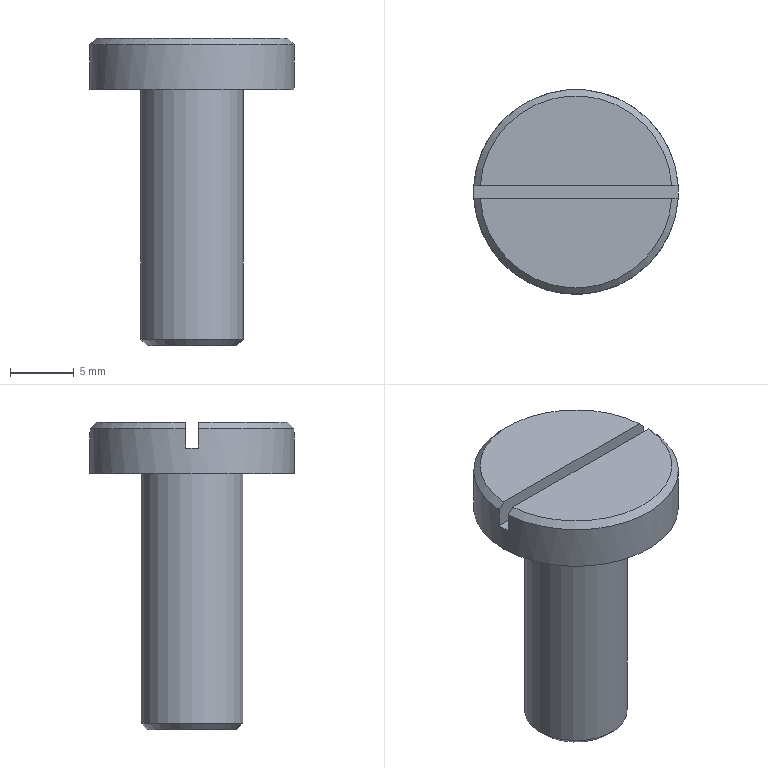Component | NX | DRILL_JIG_SCREW | 1 solid | 12 faces | box 16 x 16 x 24 mm | volume 1769 mm3 | plane 7 | cone 3 | cylinder 2 | commonest cylinder face diameters 16 x1 8 x1
STEP:
#1=CARTESIAN_POINT('',(0.,0.,0.));
#2=DIRECTION('',(0.,0.,1.));
#3=DIRECTION('',(1.,0.,0.));
#4=AXIS2_PLACEMENT_3D('',#1,#2,#3);
#5=CARTESIAN_POINT('',(-25.391,216.621,282.845));
#6=VERTEX_POINT('',#5);
#7=CARTESIAN_POINT('',(-10.425,216.621,282.845));
#8=VERTEX_POINT('',#7);
#9=CARTESIAN_POINT('',(-25.908,216.621,282.845));
#10=DIRECTION('',(1.,0.,0.));
#11=VECTOR('',#10,1.);
#12=LINE('',#9,#11);
#13=CARTESIAN_POINT('',(-17.908,216.121,282.845));
#14=DIRECTION('',(0.,0.,1.));
#15=DIRECTION('',(1.,0.,0.));
#16=AXIS2_PLACEMENT_3D('',#13,#14,#15);
#17=PLANE('',#16);
#18=CARTESIAN_POINT('',(-8.,0.5));
#19=DIRECTION('',(1.,0.));
#20=VECTOR('',#19,1.);
#21=LINE('',#18,#20);
#22=(GEOMETRIC_REPRESENTATION_CONTEXT(2)PARAMETRIC_REPRESENTATION_CONTEXT()REPRESENTATION_CONTEXT('',''));
#23=DEFINITIONAL_REPRESENTATION('',(#21),#22);
#24=PCURVE('',#17,#23);
#25=CARTESIAN_POINT('',(-25.908,216.621,282.845));
#26=DIRECTION('',(-0.,1.,0.));
#27=DIRECTION('',(1.,0.,0.));
#28=AXIS2_PLACEMENT_3D('',#25,#26,#27);
#29=PLANE('',#28);
#30=CARTESIAN_POINT('',(0.,0.));
#31=DIRECTION('',(1.,0.));
#32=VECTOR('',#31,1.);
#33=LINE('',#30,#32);
#34=(GEOMETRIC_REPRESENTATION_CONTEXT(2)PARAMETRIC_REPRESENTATION_CONTEXT()REPRESENTATION_CONTEXT('',''));
#35=DEFINITIONAL_REPRESENTATION('',(#33),#34);
#36=PCURVE('',#29,#35);
#37=SURFACE_CURVE('',#12,(#24,#36),.PCURVE_S1.);
#38=EDGE_CURVE('',#6,#8,#37,.T.);
#39=ORIENTED_EDGE('',*,*,#38,.T.);
#40=CARTESIAN_POINT('',(-17.908,216.121,282.845));
#41=DIRECTION('',(0.,0.,1.));
#42=DIRECTION('',(1.,0.,0.));
#43=AXIS2_PLACEMENT_3D('',#40,#41,#42);
#44=CIRCLE('',#43,7.5);
#45=CARTESIAN_POINT('',(0.,0.));
#46=DIRECTION('',(1.,0.));
#47=AXIS2_PLACEMENT_2D('',#45,#46);
#48=CIRCLE('',#47,7.5);
#49=(GEOMETRIC_REPRESENTATION_CONTEXT(2)PARAMETRIC_REPRESENTATION_CONTEXT()REPRESENTATION_CONTEXT('',''));
#50=DEFINITIONAL_REPRESENTATION('',(#48),#49);
#51=PCURVE('',#17,#50);
#52=CARTESIAN_POINT('',(-17.908,216.121,282.345));
#53=DIRECTION('',(0.,0.,-1.));
#54=DIRECTION('',(-1.,0.,0.));
#55=AXIS2_PLACEMENT_3D('',#52,#53,#54);
#56=CONICAL_SURFACE('',#55,8.,0.7854);
#57=CARTESIAN_POINT('',(3.142,-0.5));
#58=DIRECTION('',(-1.,0.));
#59=VECTOR('',#58,1.);
#60=LINE('',#57,#59);
#61=(GEOMETRIC_REPRESENTATION_CONTEXT(2)PARAMETRIC_REPRESENTATION_CONTEXT()REPRESENTATION_CONTEXT('',''));
#62=DEFINITIONAL_REPRESENTATION('',(#60),#61);
#63=PCURVE('',#56,#62);
#64=SURFACE_CURVE('',#44,(#51,#63),.PCURVE_S1.);
#65=EDGE_CURVE('',#8,#6,#64,.T.);
#66=ORIENTED_EDGE('',*,*,#65,.T.);
#67=EDGE_LOOP('',(#39,#66));
#68=FACE_BOUND('',#67,.T.);
#69=ADVANCED_FACE('',(#68),#17,.T.);
#70=CARTESIAN_POINT('',(-21.908,216.121,278.845));
#71=VERTEX_POINT('',#70);
#72=CARTESIAN_POINT('',(-17.908,216.121,278.845));
#73=DIRECTION('',(0.,0.,-1.));
#74=DIRECTION('',(-1.,0.,0.));
#75=AXIS2_PLACEMENT_3D('',#72,#73,#74);
#76=CIRCLE('',#75,4.);
#77=CARTESIAN_POINT('',(-17.908,216.121,278.845));
#78=DIRECTION('',(0.,0.,-1.));
#79=DIRECTION('',(-1.,0.,0.));
#80=AXIS2_PLACEMENT_3D('',#77,#78,#79);
#81=PLANE('',#80);
#82=CARTESIAN_POINT('',(0.,0.));
#83=DIRECTION('',(1.,0.));
#84=AXIS2_PLACEMENT_2D('',#82,#83);
#85=CIRCLE('',#84,4.);
#86=(GEOMETRIC_REPRESENTATION_CONTEXT(2)PARAMETRIC_REPRESENTATION_CONTEXT()REPRESENTATION_CONTEXT('',''));
#87=DEFINITIONAL_REPRESENTATION('',(#85),#86);
#88=PCURVE('',#81,#87);
#89=CARTESIAN_POINT('',(-17.908,216.121,278.845));
#90=DIRECTION('',(0.,0.,-1.));
#91=DIRECTION('',(-1.,0.,0.));
#92=AXIS2_PLACEMENT_3D('',#89,#90,#91);
#93=CYLINDRICAL_SURFACE('',#92,4.);
#94=CARTESIAN_POINT('',(0.,0.));
#95=DIRECTION('',(1.,0.));
#96=VECTOR('',#95,1.);
#97=LINE('',#94,#96);
#98=(GEOMETRIC_REPRESENTATION_CONTEXT(2)PARAMETRIC_REPRESENTATION_CONTEXT()REPRESENTATION_CONTEXT('',''));
#99=DEFINITIONAL_REPRESENTATION('',(#97),#98);
#100=PCURVE('',#93,#99);
#101=SURFACE_CURVE('',#76,(#88,#100),.PCURVE_S1.);
#102=EDGE_CURVE('',#71,#71,#101,.T.);
#103=ORIENTED_EDGE('',*,*,#102,.F.);
#104=EDGE_LOOP('',(#103));
#105=FACE_BOUND('',#104,.T.);
#106=CARTESIAN_POINT('',(-25.908,216.121,278.845));
#107=VERTEX_POINT('',#106);
#108=CARTESIAN_POINT('',(-17.908,216.121,278.845));
#109=DIRECTION('',(0.,0.,1.));
#110=DIRECTION('',(-1.,0.,0.));
#111=AXIS2_PLACEMENT_3D('',#108,#109,#110);
#112=CIRCLE('',#111,8.);
#113=CARTESIAN_POINT('',(8.,0.));
#114=CARTESIAN_POINT('',(8.,-13.856));
#115=CARTESIAN_POINT('',(-4.,-6.928));
#116=CARTESIAN_POINT('',(-16.,-0.));
#117=CARTESIAN_POINT('',(-4.,6.928));
#118=CARTESIAN_POINT('',(8.,13.856));
#119=CARTESIAN_POINT('',(8.,0.));
#120=(BOUNDED_CURVE()B_SPLINE_CURVE(2,(#113,#114,#115,#116,#117,#118,#119),.UNSPECIFIED.,.T.,.F.)B_SPLINE_CURVE_WITH_KNOTS((1,2,2,2,2,1),(-2.094,0.,2.094,4.189,6.283,8.378),.UNSPECIFIED.)CURVE()GEOMETRIC_REPRESENTATION_ITEM()RATIONAL_B_SPLINE_CURVE((1.,0.5,1.,0.5,1.,0.5,1.))REPRESENTATION_ITEM(''));
#121=(GEOMETRIC_REPRESENTATION_CONTEXT(2)PARAMETRIC_REPRESENTATION_CONTEXT()REPRESENTATION_CONTEXT('',''));
#122=DEFINITIONAL_REPRESENTATION('',(#120),#121);
#123=PCURVE('',#81,#122);
#124=CARTESIAN_POINT('',(-17.908,216.121,282.845));
#125=DIRECTION('',(0.,0.,-1.));
#126=DIRECTION('',(-1.,0.,0.));
#127=AXIS2_PLACEMENT_3D('',#124,#125,#126);
#128=CYLINDRICAL_SURFACE('',#127,8.);
#129=CARTESIAN_POINT('',(6.283,4.));
#130=DIRECTION('',(-1.,0.));
#131=VECTOR('',#130,1.);
#132=LINE('',#129,#131);
#133=(GEOMETRIC_REPRESENTATION_CONTEXT(2)PARAMETRIC_REPRESENTATION_CONTEXT()REPRESENTATION_CONTEXT('',''));
#134=DEFINITIONAL_REPRESENTATION('',(#132),#133);
#135=PCURVE('',#128,#134);
#136=SURFACE_CURVE('',#112,(#123,#135),.PCURVE_S1.);
#137=EDGE_CURVE('',#107,#107,#136,.T.);
#138=ORIENTED_EDGE('',*,*,#137,.F.);
#139=EDGE_LOOP('',(#138));
#140=FACE_BOUND('',#139,.T.);
#141=ADVANCED_FACE('',(#105,#140),#81,.T.);
#142=CARTESIAN_POINT('',(-25.391,215.621,282.845));
#143=VERTEX_POINT('',#142);
#144=CARTESIAN_POINT('',(-10.425,215.621,282.845));
#145=VERTEX_POINT('',#144);
#146=CARTESIAN_POINT('',(-25.908,215.621,282.845));
#147=DIRECTION('',(1.,0.,0.));
#148=VECTOR('',#147,1.);
#149=LINE('',#146,#148);
#150=CARTESIAN_POINT('',(-17.908,216.121,282.845));
#151=DIRECTION('',(0.,0.,1.));
#152=DIRECTION('',(1.,0.,0.));
#153=AXIS2_PLACEMENT_3D('',#150,#151,#152);
#154=PLANE('',#153);
#155=CARTESIAN_POINT('',(-8.,-0.5));
#156=DIRECTION('',(1.,0.));
#157=VECTOR('',#156,1.);
#158=LINE('',#155,#157);
#159=(GEOMETRIC_REPRESENTATION_CONTEXT(2)PARAMETRIC_REPRESENTATION_CONTEXT()REPRESENTATION_CONTEXT('',''));
#160=DEFINITIONAL_REPRESENTATION('',(#158),#159);
#161=PCURVE('',#154,#160);
#162=CARTESIAN_POINT('',(-25.908,215.621,282.845));
#163=DIRECTION('',(-0.,1.,0.));
#164=DIRECTION('',(1.,0.,0.));
#165=AXIS2_PLACEMENT_3D('',#162,#163,#164);
#166=PLANE('',#165);
#167=CARTESIAN_POINT('',(0.,0.));
#168=DIRECTION('',(1.,0.));
#169=VECTOR('',#168,1.);
#170=LINE('',#167,#169);
#171=(GEOMETRIC_REPRESENTATION_CONTEXT(2)PARAMETRIC_REPRESENTATION_CONTEXT()REPRESENTATION_CONTEXT('',''));
#172=DEFINITIONAL_REPRESENTATION('',(#170),#171);
#173=PCURVE('',#166,#172);
#174=SURFACE_CURVE('',#149,(#161,#173),.PCURVE_S1.);
#175=EDGE_CURVE('',#143,#145,#174,.T.);
#176=ORIENTED_EDGE('',*,*,#175,.F.);
#177=CARTESIAN_POINT('',(-17.908,216.121,282.845));
#178=DIRECTION('',(0.,0.,1.));
#179=DIRECTION('',(1.,0.,0.));
#180=AXIS2_PLACEMENT_3D('',#177,#178,#179);
#181=CIRCLE('',#180,7.5);
#182=CARTESIAN_POINT('',(0.,0.));
#183=DIRECTION('',(1.,0.));
#184=AXIS2_PLACEMENT_2D('',#182,#183);
#185=CIRCLE('',#184,7.5);
#186=(GEOMETRIC_REPRESENTATION_CONTEXT(2)PARAMETRIC_REPRESENTATION_CONTEXT()REPRESENTATION_CONTEXT('',''));
#187=DEFINITIONAL_REPRESENTATION('',(#185),#186);
#188=PCURVE('',#154,#187);
#189=CARTESIAN_POINT('',(-17.908,216.121,282.345));
#190=DIRECTION('',(0.,0.,-1.));
#191=DIRECTION('',(-1.,0.,0.));
#192=AXIS2_PLACEMENT_3D('',#189,#190,#191);
#193=CONICAL_SURFACE('',#192,8.,0.7854);
#194=CARTESIAN_POINT('',(9.425,-0.5));
#195=DIRECTION('',(-1.,0.));
#196=VECTOR('',#195,1.);
#197=LINE('',#194,#196);
#198=(GEOMETRIC_REPRESENTATION_CONTEXT(2)PARAMETRIC_REPRESENTATION_CONTEXT()REPRESENTATION_CONTEXT('',''));
#199=DEFINITIONAL_REPRESENTATION('',(#197),#198);
#200=PCURVE('',#193,#199);
#201=SURFACE_CURVE('',#181,(#188,#200),.PCURVE_S1.);
#202=EDGE_CURVE('',#143,#145,#201,.T.);
#203=ORIENTED_EDGE('',*,*,#202,.T.);
#204=EDGE_LOOP('',(#176,#203));
#205=FACE_BOUND('',#204,.T.);
#206=ADVANCED_FACE('',(#205),#154,.T.);
#207=CARTESIAN_POINT('',(-25.892,216.621,282.345));
#208=VERTEX_POINT('',#207);
#209=CARTESIAN_POINT('',(-25.892,216.621,280.845));
#210=VERTEX_POINT('',#209);
#211=CARTESIAN_POINT('',(-25.892,216.621,282.845));
#212=DIRECTION('',(0.,0.,-1.));
#213=VECTOR('',#212,1.);
#214=LINE('',#211,#213);
#215=CARTESIAN_POINT('',(0.06254,0.));
#216=DIRECTION('',(0.,1.));
#217=VECTOR('',#216,1.);
#218=LINE('',#215,#217);
#219=(GEOMETRIC_REPRESENTATION_CONTEXT(2)PARAMETRIC_REPRESENTATION_CONTEXT()REPRESENTATION_CONTEXT('',''));
#220=DEFINITIONAL_REPRESENTATION('',(#218),#219);
#221=PCURVE('',#128,#220);
#222=CARTESIAN_POINT('',(0.01564,0.));
#223=DIRECTION('',(0.,1.));
#224=VECTOR('',#223,1.);
#225=LINE('',#222,#224);
#226=(GEOMETRIC_REPRESENTATION_CONTEXT(2)PARAMETRIC_REPRESENTATION_CONTEXT()REPRESENTATION_CONTEXT('',''));
#227=DEFINITIONAL_REPRESENTATION('',(#225),#226);
#228=PCURVE('',#29,#227);
#229=SURFACE_CURVE('',#214,(#221,#228),.PCURVE_S1.);
#230=EDGE_CURVE('',#208,#210,#229,.T.);
#231=ORIENTED_EDGE('',*,*,#230,.F.);
#232=CARTESIAN_POINT('',(-9.924,216.621,282.345));
#233=VERTEX_POINT('',#232);
#234=CARTESIAN_POINT('',(-17.908,216.121,282.345));
#235=DIRECTION('',(0.,0.,-1.));
#236=DIRECTION('',(1.,0.,0.));
#237=AXIS2_PLACEMENT_3D('',#234,#235,#236);
#238=CIRCLE('',#237,8.);
#239=CARTESIAN_POINT('',(-3.142,0.5));
#240=DIRECTION('',(1.,0.));
#241=VECTOR('',#240,1.);
#242=LINE('',#239,#241);
#243=(GEOMETRIC_REPRESENTATION_CONTEXT(2)PARAMETRIC_REPRESENTATION_CONTEXT()REPRESENTATION_CONTEXT('',''));
#244=DEFINITIONAL_REPRESENTATION('',(#242),#243);
#245=PCURVE('',#128,#244);
#246=CARTESIAN_POINT('',(-3.142,0.));
#247=DIRECTION('',(1.,0.));
#248=VECTOR('',#247,1.);
#249=LINE('',#246,#248);
#250=(GEOMETRIC_REPRESENTATION_CONTEXT(2)PARAMETRIC_REPRESENTATION_CONTEXT()REPRESENTATION_CONTEXT('',''));
#251=DEFINITIONAL_REPRESENTATION('',(#249),#250);
#252=PCURVE('',#56,#251);
#253=SURFACE_CURVE('',#238,(#245,#252),.PCURVE_S1.);
#254=EDGE_CURVE('',#208,#233,#253,.T.);
#255=ORIENTED_EDGE('',*,*,#254,.T.);
#256=CARTESIAN_POINT('',(-9.924,216.621,280.845));
#257=VERTEX_POINT('',#256);
#258=CARTESIAN_POINT('',(-9.924,216.621,282.845));
#259=DIRECTION('',(0.,0.,1.));
#260=VECTOR('',#259,1.);
#261=LINE('',#258,#260);
#262=CARTESIAN_POINT('',(3.079,0.));
#263=DIRECTION('',(0.,-1.));
#264=VECTOR('',#263,1.);
#265=LINE('',#262,#264);
#266=(GEOMETRIC_REPRESENTATION_CONTEXT(2)PARAMETRIC_REPRESENTATION_CONTEXT()REPRESENTATION_CONTEXT('',''));
#267=DEFINITIONAL_REPRESENTATION('',(#265),#266);
#268=PCURVE('',#128,#267);
#269=CARTESIAN_POINT('',(15.984,0.));
#270=DIRECTION('',(0.,-1.));
#271=VECTOR('',#270,1.);
#272=LINE('',#269,#271);
#273=(GEOMETRIC_REPRESENTATION_CONTEXT(2)PARAMETRIC_REPRESENTATION_CONTEXT()REPRESENTATION_CONTEXT('',''));
#274=DEFINITIONAL_REPRESENTATION('',(#272),#273);
#275=PCURVE('',#29,#274);
#276=SURFACE_CURVE('',#261,(#268,#275),.PCURVE_S1.);
#277=EDGE_CURVE('',#257,#233,#276,.T.);
#278=ORIENTED_EDGE('',*,*,#277,.F.);
#279=CARTESIAN_POINT('',(-9.924,215.621,280.845));
#280=VERTEX_POINT('',#279);
#281=CARTESIAN_POINT('',(-17.908,216.121,280.845));
#282=DIRECTION('',(0.,0.,1.));
#283=DIRECTION('',(1.,0.,0.));
#284=AXIS2_PLACEMENT_3D('',#281,#282,#283);
#285=CIRCLE('',#284,8.);
#286=CARTESIAN_POINT('',(9.425,2.));
#287=DIRECTION('',(-1.,0.));
#288=VECTOR('',#287,1.);
#289=LINE('',#286,#288);
#290=(GEOMETRIC_REPRESENTATION_CONTEXT(2)PARAMETRIC_REPRESENTATION_CONTEXT()REPRESENTATION_CONTEXT('',''));
#291=DEFINITIONAL_REPRESENTATION('',(#289),#290);
#292=PCURVE('',#128,#291);
#293=CARTESIAN_POINT('',(-25.908,216.121,280.845));
#294=DIRECTION('',(0.,0.,1.));
#295=DIRECTION('',(1.,0.,0.));
#296=AXIS2_PLACEMENT_3D('',#293,#294,#295);
#297=PLANE('',#296);
#298=CARTESIAN_POINT('',(8.,-0.));
#299=DIRECTION('',(1.,-0.));
#300=AXIS2_PLACEMENT_2D('',#298,#299);
#301=CIRCLE('',#300,8.);
#302=(GEOMETRIC_REPRESENTATION_CONTEXT(2)PARAMETRIC_REPRESENTATION_CONTEXT()REPRESENTATION_CONTEXT('',''));
#303=DEFINITIONAL_REPRESENTATION('',(#301),#302);
#304=PCURVE('',#297,#303);
#305=SURFACE_CURVE('',#285,(#292,#304),.PCURVE_S1.);
#306=EDGE_CURVE('',#280,#257,#305,.T.);
#307=ORIENTED_EDGE('',*,*,#306,.F.);
#308=CARTESIAN_POINT('',(-9.924,215.621,282.345));
#309=VERTEX_POINT('',#308);
#310=CARTESIAN_POINT('',(-9.924,215.621,282.845));
#311=DIRECTION('',(0.,0.,1.));
#312=VECTOR('',#311,1.);
#313=LINE('',#310,#312);
#314=CARTESIAN_POINT('',(3.204,0.));
#315=DIRECTION('',(0.,-1.));
#316=VECTOR('',#315,1.);
#317=LINE('',#314,#316);
#318=(GEOMETRIC_REPRESENTATION_CONTEXT(2)PARAMETRIC_REPRESENTATION_CONTEXT()REPRESENTATION_CONTEXT('',''));
#319=DEFINITIONAL_REPRESENTATION('',(#317),#318);
#320=PCURVE('',#128,#319);
#321=CARTESIAN_POINT('',(15.984,0.));
#322=DIRECTION('',(0.,-1.));
#323=VECTOR('',#322,1.);
#324=LINE('',#321,#323);
#325=(GEOMETRIC_REPRESENTATION_CONTEXT(2)PARAMETRIC_REPRESENTATION_CONTEXT()REPRESENTATION_CONTEXT('',''));
#326=DEFINITIONAL_REPRESENTATION('',(#324),#325);
#327=PCURVE('',#166,#326);
#328=SURFACE_CURVE('',#313,(#320,#327),.PCURVE_S1.);
#329=EDGE_CURVE('',#280,#309,#328,.T.);
#330=ORIENTED_EDGE('',*,*,#329,.T.);
#331=CARTESIAN_POINT('',(-25.892,215.621,282.345));
#332=VERTEX_POINT('',#331);
#333=CARTESIAN_POINT('',(-17.908,216.121,282.345));
#334=DIRECTION('',(0.,0.,-1.));
#335=DIRECTION('',(1.,0.,0.));
#336=AXIS2_PLACEMENT_3D('',#333,#334,#335);
#337=CIRCLE('',#336,8.);
#338=CARTESIAN_POINT('',(3.142,0.5));
#339=DIRECTION('',(1.,0.));
#340=VECTOR('',#339,1.);
#341=LINE('',#338,#340);
#342=(GEOMETRIC_REPRESENTATION_CONTEXT(2)PARAMETRIC_REPRESENTATION_CONTEXT()REPRESENTATION_CONTEXT('',''));
#343=DEFINITIONAL_REPRESENTATION('',(#341),#342);
#344=PCURVE('',#128,#343);
#345=CARTESIAN_POINT('',(3.142,0.));
#346=DIRECTION('',(1.,0.));
#347=VECTOR('',#346,1.);
#348=LINE('',#345,#347);
#349=(GEOMETRIC_REPRESENTATION_CONTEXT(2)PARAMETRIC_REPRESENTATION_CONTEXT()REPRESENTATION_CONTEXT('',''));
#350=DEFINITIONAL_REPRESENTATION('',(#348),#349);
#351=PCURVE('',#193,#350);
#352=SURFACE_CURVE('',#337,(#344,#351),.PCURVE_S1.);
#353=EDGE_CURVE('',#309,#332,#352,.T.);
#354=ORIENTED_EDGE('',*,*,#353,.T.);
#355=CARTESIAN_POINT('',(-25.892,215.621,280.845));
#356=VERTEX_POINT('',#355);
#357=CARTESIAN_POINT('',(-25.892,215.621,282.845));
#358=DIRECTION('',(0.,0.,-1.));
#359=VECTOR('',#358,1.);
#360=LINE('',#357,#359);
#361=CARTESIAN_POINT('',(6.221,0.));
#362=DIRECTION('',(0.,1.));
#363=VECTOR('',#362,1.);
#364=LINE('',#361,#363);
#365=(GEOMETRIC_REPRESENTATION_CONTEXT(2)PARAMETRIC_REPRESENTATION_CONTEXT()REPRESENTATION_CONTEXT('',''));
#366=DEFINITIONAL_REPRESENTATION('',(#364),#365);
#367=PCURVE('',#128,#366);
#368=CARTESIAN_POINT('',(0.01564,0.));
#369=DIRECTION('',(0.,1.));
#370=VECTOR('',#369,1.);
#371=LINE('',#368,#370);
#372=(GEOMETRIC_REPRESENTATION_CONTEXT(2)PARAMETRIC_REPRESENTATION_CONTEXT()REPRESENTATION_CONTEXT('',''));
#373=DEFINITIONAL_REPRESENTATION('',(#371),#372);
#374=PCURVE('',#166,#373);
#375=SURFACE_CURVE('',#360,(#367,#374),.PCURVE_S1.);
#376=EDGE_CURVE('',#332,#356,#375,.T.);
#377=ORIENTED_EDGE('',*,*,#376,.T.);
#378=CARTESIAN_POINT('',(-25.908,216.121,280.845));
#379=VERTEX_POINT('',#378);
#380=CARTESIAN_POINT('',(-17.908,216.121,280.845));
#381=DIRECTION('',(0.,0.,1.));
#382=DIRECTION('',(1.,0.,0.));
#383=AXIS2_PLACEMENT_3D('',#380,#381,#382);
#384=CIRCLE('',#383,8.);
#385=CARTESIAN_POINT('',(9.425,2.));
#386=DIRECTION('',(-1.,0.));
#387=VECTOR('',#386,1.);
#388=LINE('',#385,#387);
#389=(GEOMETRIC_REPRESENTATION_CONTEXT(2)PARAMETRIC_REPRESENTATION_CONTEXT()REPRESENTATION_CONTEXT('',''));
#390=DEFINITIONAL_REPRESENTATION('',(#388),#389);
#391=PCURVE('',#128,#390);
#392=CARTESIAN_POINT('',(8.,-0.));
#393=DIRECTION('',(1.,-0.));
#394=AXIS2_PLACEMENT_2D('',#392,#393);
#395=CIRCLE('',#394,8.);
#396=(GEOMETRIC_REPRESENTATION_CONTEXT(2)PARAMETRIC_REPRESENTATION_CONTEXT()REPRESENTATION_CONTEXT('',''));
#397=DEFINITIONAL_REPRESENTATION('',(#395),#396);
#398=PCURVE('',#297,#397);
#399=SURFACE_CURVE('',#384,(#391,#398),.PCURVE_S1.);
#400=EDGE_CURVE('',#379,#356,#399,.T.);
#401=ORIENTED_EDGE('',*,*,#400,.F.);
#402=CARTESIAN_POINT('',(-25.908,216.121,280.845));
#403=CARTESIAN_POINT('',(-25.908,216.121,278.845));
#404=B_SPLINE_CURVE_WITH_KNOTS('',1,(#402,#403),.UNSPECIFIED.,.F.,.F.,(2,2),(2.,4.),.PIECEWISE_BEZIER_KNOTS.);
#405=CARTESIAN_POINT('',(6.283,0.));
#406=DIRECTION('',(0.,1.));
#407=VECTOR('',#406,1.);
#408=LINE('',#405,#407);
#409=(GEOMETRIC_REPRESENTATION_CONTEXT(2)PARAMETRIC_REPRESENTATION_CONTEXT()REPRESENTATION_CONTEXT('',''));
#410=DEFINITIONAL_REPRESENTATION('',(#408),#409);
#411=PCURVE('',#128,#410);
#412=CARTESIAN_POINT('',(0.,0.));
#413=DIRECTION('',(0.,1.));
#414=VECTOR('',#413,1.);
#415=LINE('',#412,#414);
#416=(GEOMETRIC_REPRESENTATION_CONTEXT(2)PARAMETRIC_REPRESENTATION_CONTEXT()REPRESENTATION_CONTEXT('',''));
#417=DEFINITIONAL_REPRESENTATION('',(#415),#416);
#418=PCURVE('',#128,#417);
#419=SEAM_CURVE('',#404,(#411,#418),.PCURVE_S1.);
#420=EDGE_CURVE('',#379,#107,#419,.T.);
#421=ORIENTED_EDGE('',*,*,#420,.T.);
#422=ORIENTED_EDGE('',*,*,#137,.T.);
#423=ORIENTED_EDGE('',*,*,#420,.F.);
#424=CARTESIAN_POINT('',(-17.908,216.121,280.845));
#425=DIRECTION('',(0.,0.,1.));
#426=DIRECTION('',(1.,0.,0.));
#427=AXIS2_PLACEMENT_3D('',#424,#425,#426);
#428=CIRCLE('',#427,8.);
#429=CARTESIAN_POINT('',(3.142,2.));
#430=DIRECTION('',(-1.,0.));
#431=VECTOR('',#430,1.);
#432=LINE('',#429,#431);
#433=(GEOMETRIC_REPRESENTATION_CONTEXT(2)PARAMETRIC_REPRESENTATION_CONTEXT()REPRESENTATION_CONTEXT('',''));
#434=DEFINITIONAL_REPRESENTATION('',(#432),#433);
#435=PCURVE('',#128,#434);
#436=CARTESIAN_POINT('',(8.,-0.));
#437=DIRECTION('',(1.,-0.));
#438=AXIS2_PLACEMENT_2D('',#436,#437);
#439=CIRCLE('',#438,8.);
#440=(GEOMETRIC_REPRESENTATION_CONTEXT(2)PARAMETRIC_REPRESENTATION_CONTEXT()REPRESENTATION_CONTEXT('',''));
#441=DEFINITIONAL_REPRESENTATION('',(#439),#440);
#442=PCURVE('',#297,#441);
#443=SURFACE_CURVE('',#428,(#435,#442),.PCURVE_S1.);
#444=EDGE_CURVE('',#210,#379,#443,.T.);
#445=ORIENTED_EDGE('',*,*,#444,.F.);
#446=EDGE_LOOP('',(#231,#255,#278,#307,#330,#354,#377,#401,#421,#422,#423,#445));
#447=FACE_BOUND('',#446,.T.);
#448=ADVANCED_FACE('',(#447),#128,.T.);
#449=CARTESIAN_POINT('',(-21.408,216.121,258.845));
#450=VERTEX_POINT('',#449);
#451=CARTESIAN_POINT('',(-17.908,216.121,258.845));
#452=DIRECTION('',(0.,0.,-1.));
#453=DIRECTION('',(-1.,0.,0.));
#454=AXIS2_PLACEMENT_3D('',#451,#452,#453);
#455=CIRCLE('',#454,3.5);
#456=CARTESIAN_POINT('',(-17.908,216.121,258.845));
#457=DIRECTION('',(0.,0.,-1.));
#458=DIRECTION('',(-1.,0.,0.));
#459=AXIS2_PLACEMENT_3D('',#456,#457,#458);
#460=PLANE('',#459);
#461=CARTESIAN_POINT('',(0.,0.));
#462=DIRECTION('',(1.,0.));
#463=AXIS2_PLACEMENT_2D('',#461,#462);
#464=CIRCLE('',#463,3.5);
#465=(GEOMETRIC_REPRESENTATION_CONTEXT(2)PARAMETRIC_REPRESENTATION_CONTEXT()REPRESENTATION_CONTEXT('',''));
#466=DEFINITIONAL_REPRESENTATION('',(#464),#465);
#467=PCURVE('',#460,#466);
#468=CARTESIAN_POINT('',(-17.908,216.121,259.345));
#469=DIRECTION('',(0.,0.,1.));
#470=DIRECTION('',(1.,0.,0.));
#471=AXIS2_PLACEMENT_3D('',#468,#469,#470);
#472=CONICAL_SURFACE('',#471,4.,0.7854);
#473=CARTESIAN_POINT('',(9.425,-0.5));
#474=DIRECTION('',(-1.,0.));
#475=VECTOR('',#474,1.);
#476=LINE('',#473,#475);
#477=(GEOMETRIC_REPRESENTATION_CONTEXT(2)PARAMETRIC_REPRESENTATION_CONTEXT()REPRESENTATION_CONTEXT('',''));
#478=DEFINITIONAL_REPRESENTATION('',(#476),#477);
#479=PCURVE('',#472,#478);
#480=SURFACE_CURVE('',#455,(#467,#479),.PCURVE_S1.);
#481=EDGE_CURVE('',#450,#450,#480,.T.);
#482=ORIENTED_EDGE('',*,*,#481,.T.);
#483=EDGE_LOOP('',(#482));
#484=FACE_BOUND('',#483,.T.);
#485=ADVANCED_FACE('',(#484),#460,.T.);
#486=CARTESIAN_POINT('',(-21.908,216.121,259.345));
#487=VERTEX_POINT('',#486);
#488=CARTESIAN_POINT('',(-17.908,216.121,259.345));
#489=DIRECTION('',(0.,0.,1.));
#490=DIRECTION('',(-1.,0.,0.));
#491=AXIS2_PLACEMENT_3D('',#488,#489,#490);
#492=CIRCLE('',#491,4.);
#493=CARTESIAN_POINT('',(6.283,19.5));
#494=DIRECTION('',(-1.,0.));
#495=VECTOR('',#494,1.);
#496=LINE('',#493,#495);
#497=(GEOMETRIC_REPRESENTATION_CONTEXT(2)PARAMETRIC_REPRESENTATION_CONTEXT()REPRESENTATION_CONTEXT('',''));
#498=DEFINITIONAL_REPRESENTATION('',(#496),#497);
#499=PCURVE('',#93,#498);
#500=CARTESIAN_POINT('',(3.142,0.));
#501=DIRECTION('',(1.,0.));
#502=VECTOR('',#501,1.);
#503=LINE('',#500,#502);
#504=(GEOMETRIC_REPRESENTATION_CONTEXT(2)PARAMETRIC_REPRESENTATION_CONTEXT()REPRESENTATION_CONTEXT('',''));
#505=DEFINITIONAL_REPRESENTATION('',(#503),#504);
#506=PCURVE('',#472,#505);
#507=SURFACE_CURVE('',#492,(#499,#506),.PCURVE_S1.);
#508=EDGE_CURVE('',#487,#487,#507,.T.);
#509=ORIENTED_EDGE('',*,*,#508,.T.);
#510=CARTESIAN_POINT('',(-21.908,216.121,278.845));
#511=CARTESIAN_POINT('',(-21.908,216.121,259.345));
#512=B_SPLINE_CURVE_WITH_KNOTS('',1,(#510,#511),.UNSPECIFIED.,.F.,.F.,(2,2),(0.,19.5),.PIECEWISE_BEZIER_KNOTS.);
#513=CARTESIAN_POINT('',(0.,0.));
#514=DIRECTION('',(0.,1.));
#515=VECTOR('',#514,1.);
#516=LINE('',#513,#515);
#517=(GEOMETRIC_REPRESENTATION_CONTEXT(2)PARAMETRIC_REPRESENTATION_CONTEXT()REPRESENTATION_CONTEXT('',''));
#518=DEFINITIONAL_REPRESENTATION('',(#516),#517);
#519=PCURVE('',#93,#518);
#520=CARTESIAN_POINT('',(6.283,0.));
#521=DIRECTION('',(0.,1.));
#522=VECTOR('',#521,1.);
#523=LINE('',#520,#522);
#524=(GEOMETRIC_REPRESENTATION_CONTEXT(2)PARAMETRIC_REPRESENTATION_CONTEXT()REPRESENTATION_CONTEXT('',''));
#525=DEFINITIONAL_REPRESENTATION('',(#523),#524);
#526=PCURVE('',#93,#525);
#527=SEAM_CURVE('',#512,(#519,#526),.PCURVE_S1.);
#528=EDGE_CURVE('',#71,#487,#527,.T.);
#529=ORIENTED_EDGE('',*,*,#528,.F.);
#530=ORIENTED_EDGE('',*,*,#102,.T.);
#531=ORIENTED_EDGE('',*,*,#528,.T.);
#532=EDGE_LOOP('',(#509,#529,#530,#531));
#533=FACE_BOUND('',#532,.T.);
#534=ADVANCED_FACE('',(#533),#93,.T.);
#535=CARTESIAN_POINT('',(-25.908,216.621,280.845));
#536=DIRECTION('',(-1.,-0.,0.));
#537=VECTOR('',#536,1.);
#538=LINE('',#535,#537);
#539=CARTESIAN_POINT('',(0.,0.5));
#540=DIRECTION('',(-1.,-0.));
#541=VECTOR('',#540,1.);
#542=LINE('',#539,#541);
#543=(GEOMETRIC_REPRESENTATION_CONTEXT(2)PARAMETRIC_REPRESENTATION_CONTEXT()REPRESENTATION_CONTEXT('',''));
#544=DEFINITIONAL_REPRESENTATION('',(#542),#543);
#545=PCURVE('',#297,#544);
#546=CARTESIAN_POINT('',(0.,2.));
#547=DIRECTION('',(-1.,0.));
#548=VECTOR('',#547,1.);
#549=LINE('',#546,#548);
#550=(GEOMETRIC_REPRESENTATION_CONTEXT(2)PARAMETRIC_REPRESENTATION_CONTEXT()REPRESENTATION_CONTEXT('',''));
#551=DEFINITIONAL_REPRESENTATION('',(#549),#550);
#552=PCURVE('',#29,#551);
#553=SURFACE_CURVE('',#538,(#545,#552),.PCURVE_S1.);
#554=EDGE_CURVE('',#257,#210,#553,.T.);
#555=ORIENTED_EDGE('',*,*,#554,.T.);
#556=ORIENTED_EDGE('',*,*,#444,.T.);
#557=ORIENTED_EDGE('',*,*,#400,.T.);
#558=CARTESIAN_POINT('',(-25.908,215.621,280.845));
#559=DIRECTION('',(-1.,-0.,0.));
#560=VECTOR('',#559,1.);
#561=LINE('',#558,#560);
#562=CARTESIAN_POINT('',(-0.,-0.5));
#563=DIRECTION('',(-1.,-0.));
#564=VECTOR('',#563,1.);
#565=LINE('',#562,#564);
#566=(GEOMETRIC_REPRESENTATION_CONTEXT(2)PARAMETRIC_REPRESENTATION_CONTEXT()REPRESENTATION_CONTEXT('',''));
#567=DEFINITIONAL_REPRESENTATION('',(#565),#566);
#568=PCURVE('',#297,#567);
#569=CARTESIAN_POINT('',(0.,2.));
#570=DIRECTION('',(-1.,0.));
#571=VECTOR('',#570,1.);
#572=LINE('',#569,#571);
#573=(GEOMETRIC_REPRESENTATION_CONTEXT(2)PARAMETRIC_REPRESENTATION_CONTEXT()REPRESENTATION_CONTEXT('',''));
#574=DEFINITIONAL_REPRESENTATION('',(#572),#573);
#575=PCURVE('',#166,#574);
#576=SURFACE_CURVE('',#561,(#568,#575),.PCURVE_S1.);
#577=EDGE_CURVE('',#280,#356,#576,.T.);
#578=ORIENTED_EDGE('',*,*,#577,.F.);
#579=ORIENTED_EDGE('',*,*,#306,.T.);
#580=EDGE_LOOP('',(#555,#556,#557,#578,#579));
#581=FACE_BOUND('',#580,.T.);
#582=ADVANCED_FACE('',(#581),#297,.T.);
#583=ORIENTED_EDGE('',*,*,#277,.T.);
#584=CARTESIAN_POINT('',(-9.924,216.621,282.345));
#585=CARTESIAN_POINT('',(-10.091,216.621,282.511));
#586=CARTESIAN_POINT('',(-10.258,216.621,282.678));
#587=CARTESIAN_POINT('',(-10.425,216.621,282.845));
#588=B_SPLINE_CURVE_WITH_KNOTS('',3,(#584,#585,#586,#587),.UNSPECIFIED.,.F.,.F.,(4,4),(0.,1.),.PIECEWISE_BEZIER_KNOTS.);
#589=CARTESIAN_POINT('',(15.984,0.5));
#590=CARTESIAN_POINT('',(15.817,0.3333));
#591=CARTESIAN_POINT('',(15.65,0.1667));
#592=CARTESIAN_POINT('',(15.483,0.));
#593=B_SPLINE_CURVE_WITH_KNOTS('',3,(#589,#590,#591,#592),.UNSPECIFIED.,.F.,.F.,(4,4),(0.,1.),.PIECEWISE_BEZIER_KNOTS.);
#594=(GEOMETRIC_REPRESENTATION_CONTEXT(2)PARAMETRIC_REPRESENTATION_CONTEXT()REPRESENTATION_CONTEXT('',''));
#595=DEFINITIONAL_REPRESENTATION('',(#593),#594);
#596=PCURVE('',#29,#595);
#597=CARTESIAN_POINT('',(3.079,-0.));
#598=CARTESIAN_POINT('',(3.075,-0.5));
#599=B_SPLINE_CURVE_WITH_KNOTS('',1,(#597,#598),.UNSPECIFIED.,.F.,.F.,(2,2),(0.,1.),.PIECEWISE_BEZIER_KNOTS.);
#600=(GEOMETRIC_REPRESENTATION_CONTEXT(2)PARAMETRIC_REPRESENTATION_CONTEXT()REPRESENTATION_CONTEXT('',''));
#601=DEFINITIONAL_REPRESENTATION('',(#599),#600);
#602=PCURVE('',#56,#601);
#603=SURFACE_CURVE('',#588,(#596,#602),.PCURVE_S1.);
#604=EDGE_CURVE('',#233,#8,#603,.T.);
#605=ORIENTED_EDGE('',*,*,#604,.T.);
#606=ORIENTED_EDGE('',*,*,#38,.F.);
#607=CARTESIAN_POINT('',(-25.391,216.621,282.845));
#608=CARTESIAN_POINT('',(-25.558,216.621,282.678));
#609=CARTESIAN_POINT('',(-25.725,216.621,282.511));
#610=CARTESIAN_POINT('',(-25.892,216.621,282.345));
#611=B_SPLINE_CURVE_WITH_KNOTS('',3,(#607,#608,#609,#610),.UNSPECIFIED.,.F.,.F.,(4,4),(0.,1.),.PIECEWISE_BEZIER_KNOTS.);
#612=CARTESIAN_POINT('',(0.5167,0.));
#613=CARTESIAN_POINT('',(0.3497,0.1667));
#614=CARTESIAN_POINT('',(0.1826,0.3333));
#615=CARTESIAN_POINT('',(0.01564,0.5));
#616=B_SPLINE_CURVE_WITH_KNOTS('',3,(#612,#613,#614,#615),.UNSPECIFIED.,.F.,.F.,(4,4),(0.,1.),.PIECEWISE_BEZIER_KNOTS.);
#617=(GEOMETRIC_REPRESENTATION_CONTEXT(2)PARAMETRIC_REPRESENTATION_CONTEXT()REPRESENTATION_CONTEXT('',''));
#618=DEFINITIONAL_REPRESENTATION('',(#616),#617);
#619=PCURVE('',#29,#618);
#620=CARTESIAN_POINT('',(0.06672,-0.5));
#621=CARTESIAN_POINT('',(0.06254,0.));
#622=B_SPLINE_CURVE_WITH_KNOTS('',1,(#620,#621),.UNSPECIFIED.,.F.,.F.,(2,2),(0.,1.),.PIECEWISE_BEZIER_KNOTS.);
#623=(GEOMETRIC_REPRESENTATION_CONTEXT(2)PARAMETRIC_REPRESENTATION_CONTEXT()REPRESENTATION_CONTEXT('',''));
#624=DEFINITIONAL_REPRESENTATION('',(#622),#623);
#625=PCURVE('',#56,#624);
#626=SURFACE_CURVE('',#611,(#619,#625),.PCURVE_S1.);
#627=EDGE_CURVE('',#6,#208,#626,.T.);
#628=ORIENTED_EDGE('',*,*,#627,.T.);
#629=ORIENTED_EDGE('',*,*,#230,.T.);
#630=ORIENTED_EDGE('',*,*,#554,.F.);
#631=EDGE_LOOP('',(#583,#605,#606,#628,#629,#630));
#632=FACE_BOUND('',#631,.T.);
#633=ADVANCED_FACE('',(#632),#29,.F.);
#634=ORIENTED_EDGE('',*,*,#376,.F.);
#635=CARTESIAN_POINT('',(-25.892,215.621,282.345));
#636=CARTESIAN_POINT('',(-25.725,215.621,282.511));
#637=CARTESIAN_POINT('',(-25.558,215.621,282.678));
#638=CARTESIAN_POINT('',(-25.391,215.621,282.845));
#639=B_SPLINE_CURVE_WITH_KNOTS('',3,(#635,#636,#637,#638),.UNSPECIFIED.,.F.,.F.,(4,4),(0.,1.),.PIECEWISE_BEZIER_KNOTS.);
#640=CARTESIAN_POINT('',(0.01564,0.5));
#641=CARTESIAN_POINT('',(0.1826,0.3333));
#642=CARTESIAN_POINT('',(0.3497,0.1667));
#643=CARTESIAN_POINT('',(0.5167,0.));
#644=B_SPLINE_CURVE_WITH_KNOTS('',3,(#640,#641,#642,#643),.UNSPECIFIED.,.F.,.F.,(4,4),(0.,1.),.PIECEWISE_BEZIER_KNOTS.);
#645=(GEOMETRIC_REPRESENTATION_CONTEXT(2)PARAMETRIC_REPRESENTATION_CONTEXT()REPRESENTATION_CONTEXT('',''));
#646=DEFINITIONAL_REPRESENTATION('',(#644),#645);
#647=PCURVE('',#166,#646);
#648=CARTESIAN_POINT('',(6.221,0.));
#649=CARTESIAN_POINT('',(6.216,-0.5));
#650=B_SPLINE_CURVE_WITH_KNOTS('',1,(#648,#649),.UNSPECIFIED.,.F.,.F.,(2,2),(0.,1.),.PIECEWISE_BEZIER_KNOTS.);
#651=(GEOMETRIC_REPRESENTATION_CONTEXT(2)PARAMETRIC_REPRESENTATION_CONTEXT()REPRESENTATION_CONTEXT('',''));
#652=DEFINITIONAL_REPRESENTATION('',(#650),#651);
#653=PCURVE('',#193,#652);
#654=SURFACE_CURVE('',#639,(#647,#653),.PCURVE_S1.);
#655=EDGE_CURVE('',#332,#143,#654,.T.);
#656=ORIENTED_EDGE('',*,*,#655,.T.);
#657=ORIENTED_EDGE('',*,*,#175,.T.);
#658=CARTESIAN_POINT('',(-10.425,215.621,282.845));
#659=CARTESIAN_POINT('',(-10.258,215.621,282.678));
#660=CARTESIAN_POINT('',(-10.091,215.621,282.511));
#661=CARTESIAN_POINT('',(-9.924,215.621,282.345));
#662=B_SPLINE_CURVE_WITH_KNOTS('',3,(#658,#659,#660,#661),.UNSPECIFIED.,.F.,.F.,(4,4),(0.,1.),.PIECEWISE_BEZIER_KNOTS.);
#663=CARTESIAN_POINT('',(15.483,0.));
#664=CARTESIAN_POINT('',(15.65,0.1667));
#665=CARTESIAN_POINT('',(15.817,0.3333));
#666=CARTESIAN_POINT('',(15.984,0.5));
#667=B_SPLINE_CURVE_WITH_KNOTS('',3,(#663,#664,#665,#666),.UNSPECIFIED.,.F.,.F.,(4,4),(0.,1.),.PIECEWISE_BEZIER_KNOTS.);
#668=(GEOMETRIC_REPRESENTATION_CONTEXT(2)PARAMETRIC_REPRESENTATION_CONTEXT()REPRESENTATION_CONTEXT('',''));
#669=DEFINITIONAL_REPRESENTATION('',(#667),#668);
#670=PCURVE('',#166,#669);
#671=CARTESIAN_POINT('',(3.208,-0.5));
#672=CARTESIAN_POINT('',(3.204,-0.));
#673=B_SPLINE_CURVE_WITH_KNOTS('',1,(#671,#672),.UNSPECIFIED.,.F.,.F.,(2,2),(0.,1.),.PIECEWISE_BEZIER_KNOTS.);
#674=(GEOMETRIC_REPRESENTATION_CONTEXT(2)PARAMETRIC_REPRESENTATION_CONTEXT()REPRESENTATION_CONTEXT('',''));
#675=DEFINITIONAL_REPRESENTATION('',(#673),#674);
#676=PCURVE('',#193,#675);
#677=SURFACE_CURVE('',#662,(#670,#676),.PCURVE_S1.);
#678=EDGE_CURVE('',#145,#309,#677,.T.);
#679=ORIENTED_EDGE('',*,*,#678,.T.);
#680=ORIENTED_EDGE('',*,*,#329,.F.);
#681=ORIENTED_EDGE('',*,*,#577,.T.);
#682=EDGE_LOOP('',(#634,#656,#657,#679,#680,#681));
#683=FACE_BOUND('',#682,.T.);
#684=ADVANCED_FACE('',(#683),#166,.T.);
#685=ORIENTED_EDGE('',*,*,#627,.F.);
#686=ORIENTED_EDGE('',*,*,#65,.F.);
#687=ORIENTED_EDGE('',*,*,#604,.F.);
#688=ORIENTED_EDGE('',*,*,#254,.F.);
#689=EDGE_LOOP('',(#685,#686,#687,#688));
#690=FACE_BOUND('',#689,.T.);
#691=ADVANCED_FACE('',(#690),#56,.T.);
#692=ORIENTED_EDGE('',*,*,#678,.F.);
#693=ORIENTED_EDGE('',*,*,#202,.F.);
#694=ORIENTED_EDGE('',*,*,#655,.F.);
#695=ORIENTED_EDGE('',*,*,#353,.F.);
#696=EDGE_LOOP('',(#692,#693,#694,#695));
#697=FACE_BOUND('',#696,.T.);
#698=ADVANCED_FACE('',(#697),#193,.T.);
#699=ORIENTED_EDGE('',*,*,#481,.F.);
#700=CARTESIAN_POINT('',(-21.408,216.121,258.845));
#701=CARTESIAN_POINT('',(-21.908,216.121,259.345));
#702=B_SPLINE_CURVE_WITH_KNOTS('',1,(#700,#701),.UNSPECIFIED.,.F.,.F.,(2,2),(-0.7071,0.),.PIECEWISE_BEZIER_KNOTS.);
#703=CARTESIAN_POINT('',(9.425,0.));
#704=DIRECTION('',(0.,1.));
#705=VECTOR('',#704,1.);
#706=LINE('',#703,#705);
#707=(GEOMETRIC_REPRESENTATION_CONTEXT(2)PARAMETRIC_REPRESENTATION_CONTEXT()REPRESENTATION_CONTEXT('',''));
#708=DEFINITIONAL_REPRESENTATION('',(#706),#707);
#709=PCURVE('',#472,#708);
#710=CARTESIAN_POINT('',(3.142,0.));
#711=DIRECTION('',(0.,1.));
#712=VECTOR('',#711,1.);
#713=LINE('',#710,#712);
#714=(GEOMETRIC_REPRESENTATION_CONTEXT(2)PARAMETRIC_REPRESENTATION_CONTEXT()REPRESENTATION_CONTEXT('',''));
#715=DEFINITIONAL_REPRESENTATION('',(#713),#714);
#716=PCURVE('',#472,#715);
#717=SEAM_CURVE('',#702,(#709,#716),.PCURVE_S1.);
#718=EDGE_CURVE('',#450,#487,#717,.T.);
#719=ORIENTED_EDGE('',*,*,#718,.T.);
#720=ORIENTED_EDGE('',*,*,#508,.F.);
#721=ORIENTED_EDGE('',*,*,#718,.F.);
#722=EDGE_LOOP('',(#699,#719,#720,#721));
#723=FACE_BOUND('',#722,.T.);
#724=ADVANCED_FACE('',(#723),#472,.T.);
#725=CLOSED_SHELL('',(#69,#141,#206,#448,#485,#534,#582,#633,#684,#691,#698,#724));
#726=MANIFOLD_SOLID_BREP('',#725);
#727=(LENGTH_UNIT()NAMED_UNIT(*)SI_UNIT(.MILLI.,.METRE.));
#728=UNCERTAINTY_MEASURE_WITH_UNIT(LENGTH_MEASURE(0.0002),#727,'','');
#729=(NAMED_UNIT(*)PLANE_ANGLE_UNIT()SI_UNIT($,.RADIAN.));
#730=(NAMED_UNIT(*)SI_UNIT($,.STERADIAN.)SOLID_ANGLE_UNIT());
#731=(GEOMETRIC_REPRESENTATION_CONTEXT(3)GLOBAL_UNCERTAINTY_ASSIGNED_CONTEXT((#728))GLOBAL_UNIT_ASSIGNED_CONTEXT((#727,#729,#730))REPRESENTATION_CONTEXT('',''));
#732=ADVANCED_BREP_SHAPE_REPRESENTATION('',(#4,#726),#731);